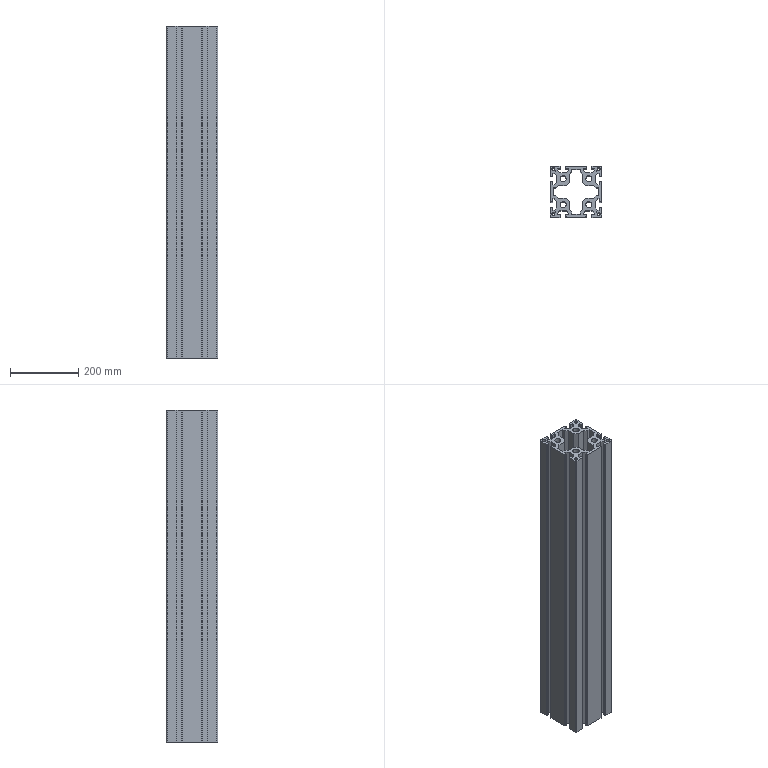Component | SolidWorks | AluminumProfile3-2 | 1 solid | 186 faces | box 150 x 150 x 970 mm | volume 8987483 mm3 | plane 162 | cylinder 24 | commonest cylinder face diameters 9 x12 18 x8 7.5 x4
build123d program:
from build123d import *

# Parameters (mm, degrees)
SKETCH1_R           = 6
BOSS_EXTRUDE1_DEPTH = 646.667
SCALE1_SCALE        = 1.5


with BuildPart() as part:
    # Sketch1 → Boss-Extrude1 (new body)
    with BuildSketch(Plane(origin=(-310, 0, 0), x_dir=(0, -1, 0), z_dir=(-1, 0, 0))):
        with BuildLine():
            Line((45, 19.9), (45, 14))
            Line((45, 14), (41.657, 14))
            Line((41.657, 14), (37.2, 18.457))
            Line((37.2, 18.457), (37.2, 31.543))
            Line((37.2, 31.543), (41.657, 36))
            Line((41.657, 36), (45, 36))
            Line((45, 36), (45, 30.1))
            Line((45, 30.1), (49, 30.1))
            Line((49, 30.1), (49, 31.1))
            Line((49, 31.1), (50, 31.1))
            Line((50, 31.1), (50, 47.5))
            ThreePointArc((50, 47.5), (49.268, 49.268), (47.5, 50))
            Line((47.5, 50), (31.1, 50))
            Line((31.1, 50), (31.1, 49))
            Line((31.1, 49), (30.1, 49))
            Line((30.1, 49), (30.1, 45))
            Line((30.1, 45), (36, 45))
            Line((36, 45), (36, 41.657))
            Line((36, 41.657), (31.543, 37.2))
            Line((31.543, 37.2), (18.457, 37.2))
            Line((18.457, 37.2), (14, 41.657))
            Line((14, 41.657), (14, 45))
            Line((14, 45), (19.9, 45))
            Line((19.9, 45), (19.9, 49))
            Line((19.9, 49), (18.9, 49))
            Line((18.9, 49), (18.9, 50))
            Line((18.9, 50), (-18.9, 50))
            Line((-18.9, 50), (-18.9, 49))
            Line((-18.9, 49), (-19.9, 49))
            Line((-19.9, 49), (-19.9, 45))
            Line((-19.9, 45), (-14, 45))
            Line((-14, 45), (-14, 41.657))
            Line((-14, 41.657), (-18.457, 37.2))
            Line((-18.457, 37.2), (-31.543, 37.2))
            Line((-31.543, 37.2), (-36, 41.657))
            Line((-36, 41.657), (-36, 45))
            Line((-36, 45), (-30.1, 45))
            Line((-30.1, 45), (-30.1, 49))
            Line((-30.1, 49), (-31.1, 49))
            Line((-31.1, 49), (-31.1, 50))
            Line((-31.1, 50), (-47.5, 50))
            ThreePointArc((-47.5, 50), (-49.268, 49.268), (-50, 47.5))
            Line((-50, 47.5), (-50, 31.1))
            Line((-50, 31.1), (-49, 31.1))
            Line((-49, 31.1), (-49, 30.1))
            Line((-49, 30.1), (-45, 30.1))
            Line((-45, 30.1), (-45, 36))
            Line((-45, 36), (-41.657, 36))
            Line((-41.657, 36), (-37.2, 31.543))
            Line((-37.2, 31.543), (-37.2, 18.457))
            Line((-37.2, 18.457), (-41.657, 14))
            Line((-41.657, 14), (-45, 14))
            Line((-45, 14), (-45, 19.9))
            Line((-45, 19.9), (-49, 19.9))
            Line((-49, 19.9), (-49, 18.9))
            Line((-49, 18.9), (-50, 18.9))
            Line((-50, 18.9), (-50, -18.9))
            Line((-50, -18.9), (-49, -18.9))
            Line((-49, -18.9), (-49, -19.9))
            Line((-49, -19.9), (-45, -19.9))
            Line((-45, -19.9), (-45, -14))
            Line((-45, -14), (-41.657, -14))
            Line((-41.657, -14), (-37.2, -18.457))
            Line((-37.2, -18.457), (-37.2, -31.543))
            Line((-37.2, -31.543), (-41.657, -36))
            Line((-41.657, -36), (-45, -36))
            Line((-45, -36), (-45, -30.1))
            Line((-45, -30.1), (-49, -30.1))
            Line((-49, -30.1), (-49, -31.1))
            Line((-49, -31.1), (-50, -31.1))
            Line((-50, -31.1), (-50, -47.5))
            ThreePointArc((-50, -47.5), (-49.268, -49.268), (-47.5, -50))
            Line((-47.5, -50), (-31.1, -50))
            Line((-31.1, -50), (-31.1, -49))
            Line((-31.1, -49), (-30.1, -49))
            Line((-30.1, -49), (-30.1, -45))
            Line((-30.1, -45), (-36, -45))
            Line((-36, -45), (-36, -41.657))
            Line((-36, -41.657), (-31.543, -37.2))
            Line((-31.543, -37.2), (-18.457, -37.2))
            Line((-18.457, -37.2), (-14, -41.657))
            Line((-14, -41.657), (-14, -45))
            Line((-14, -45), (-19.9, -45))
            Line((-19.9, -45), (-19.9, -49))
            Line((-19.9, -49), (-18.9, -49))
            Line((-18.9, -49), (-18.9, -50))
            Line((-18.9, -50), (18.9, -50))
            Line((18.9, -50), (18.9, -49))
            Line((18.9, -49), (19.9, -49))
            Line((19.9, -49), (19.9, -45))
            Line((19.9, -45), (14, -45))
            Line((14, -45), (14, -41.657))
            Line((14, -41.657), (18.457, -37.2))
            Line((18.457, -37.2), (31.543, -37.2))
            Line((31.543, -37.2), (36, -41.657))
            Line((36, -41.657), (36, -45))
            Line((36, -45), (30.1, -45))
            Line((30.1, -45), (30.1, -49))
            Line((30.1, -49), (31.1, -49))
            Line((31.1, -49), (31.1, -50))
            Line((31.1, -50), (47.5, -50))
            ThreePointArc((47.5, -50), (49.268, -49.268), (50, -47.5))
            Line((50, -47.5), (50, -31.1))
            Line((50, -31.1), (49, -31.1))
            Line((49, -31.1), (49, -30.1))
            Line((49, -30.1), (45, -30.1))
            Line((45, -30.1), (45, -36))
            Line((45, -36), (41.657, -36))
            Line((41.657, -36), (37.2, -31.543))
            Line((37.2, -31.543), (37.2, -18.457))
            Line((37.2, -18.457), (41.657, -14))
            Line((41.657, -14), (45, -14))
            Line((45, -14), (45, -19.9))
            Line((45, -19.9), (49, -19.9))
            Line((49, -19.9), (49, -18.9))
            Line((49, -18.9), (50, -18.9))
            Line((50, -18.9), (50, 18.9))
            Line((50, 18.9), (49, 18.9))
            Line((49, 18.9), (49, 19.9))
            Line((49, 19.9), (45, 19.9))
        make_face()
        with Locations(Location((25, 25, 0), (0, 0, 180))):
            Circle(SKETCH1_R, mode=Mode.SUBTRACT)
        with Locations(Location((25, -25, 0), (0, 0, 180))):
            Circle(SKETCH1_R, mode=Mode.SUBTRACT)
        with Locations(Location((-25, 25, 0), (0, 0, 180))):
            Circle(SKETCH1_R, mode=Mode.SUBTRACT)
        with Locations(Location((-25, -25, 0), (0, 0, 180))):
            Circle(SKETCH1_R, mode=Mode.SUBTRACT)
        with BuildLine():
            Line((38.981, -40.678), (40.678, -38.981))
            Line((40.678, -38.981), (42.904, -41.207))
            ThreePointArc((42.904, -41.207), (46.121, -46.121), (41.207, -42.904))
            Line((41.207, -42.904), (38.981, -40.678))
        make_face(mode=Mode.SUBTRACT)
        with BuildLine():
            Line((-40.678, -38.981), (-38.981, -40.678))
            Line((-38.981, -40.678), (-41.207, -42.904))
            ThreePointArc((-41.207, -42.904), (-46.121, -46.121), (-42.904, -41.207))
            Line((-42.904, -41.207), (-40.678, -38.981))
        make_face(mode=Mode.SUBTRACT)
        Polygon((34.372, 12.8), (39.172, 8), (44, 8), (44, -8), (39.172, -8), (34.372, -12.8), (18.8, -12.8), (12.8, -18.8), (12.8, -34.372), (8, -39.172), (8, -44), (-8, -44), (-8, -39.172), (-12.8, -34.372), (-12.8, -18.8), (-18.8, -12.8), (-34.372, -12.8), (-39.172, -8), (-44, -8), (-44, 8), (-39.172, 8), (-34.372, 12.8), (-18.8, 12.8), (-12.8, 18.8), (-12.8, 34.372), (-8, 39.172), (-8, 44), (8, 44), (8, 39.172), (12.8, 34.372), (12.8, 18.8), (18.8, 12.8), align=None, mode=Mode.SUBTRACT)
        with BuildLine():
            Line((42.904, 41.207), (40.678, 38.981))
            Line((40.678, 38.981), (38.981, 40.678))
            Line((38.981, 40.678), (41.207, 42.904))
            ThreePointArc((41.207, 42.904), (46.121, 46.121), (42.904, 41.207))
        make_face(mode=Mode.SUBTRACT)
        with BuildLine():
            Line((-41.207, 42.904), (-38.981, 40.678))
            Line((-38.981, 40.678), (-40.678, 38.981))
            Line((-40.678, 38.981), (-42.904, 41.207))
            ThreePointArc((-42.904, 41.207), (-46.121, 46.121), (-41.207, 42.904))
        make_face(mode=Mode.SUBTRACT)
    extrude(amount=-BOSS_EXTRUDE1_DEPTH)


with BuildPart() as part_1:
    # Scale1: scaled about (13.333, 0, -0)
    add(part.part.scale(SCALE1_SCALE).moved(Location((-6.667, 0, 0))))


solid = part_1.part

# Placed as in the assembly
solid = solid.moved(Location((-15, -956, 508.333), (0, 90, 0)))